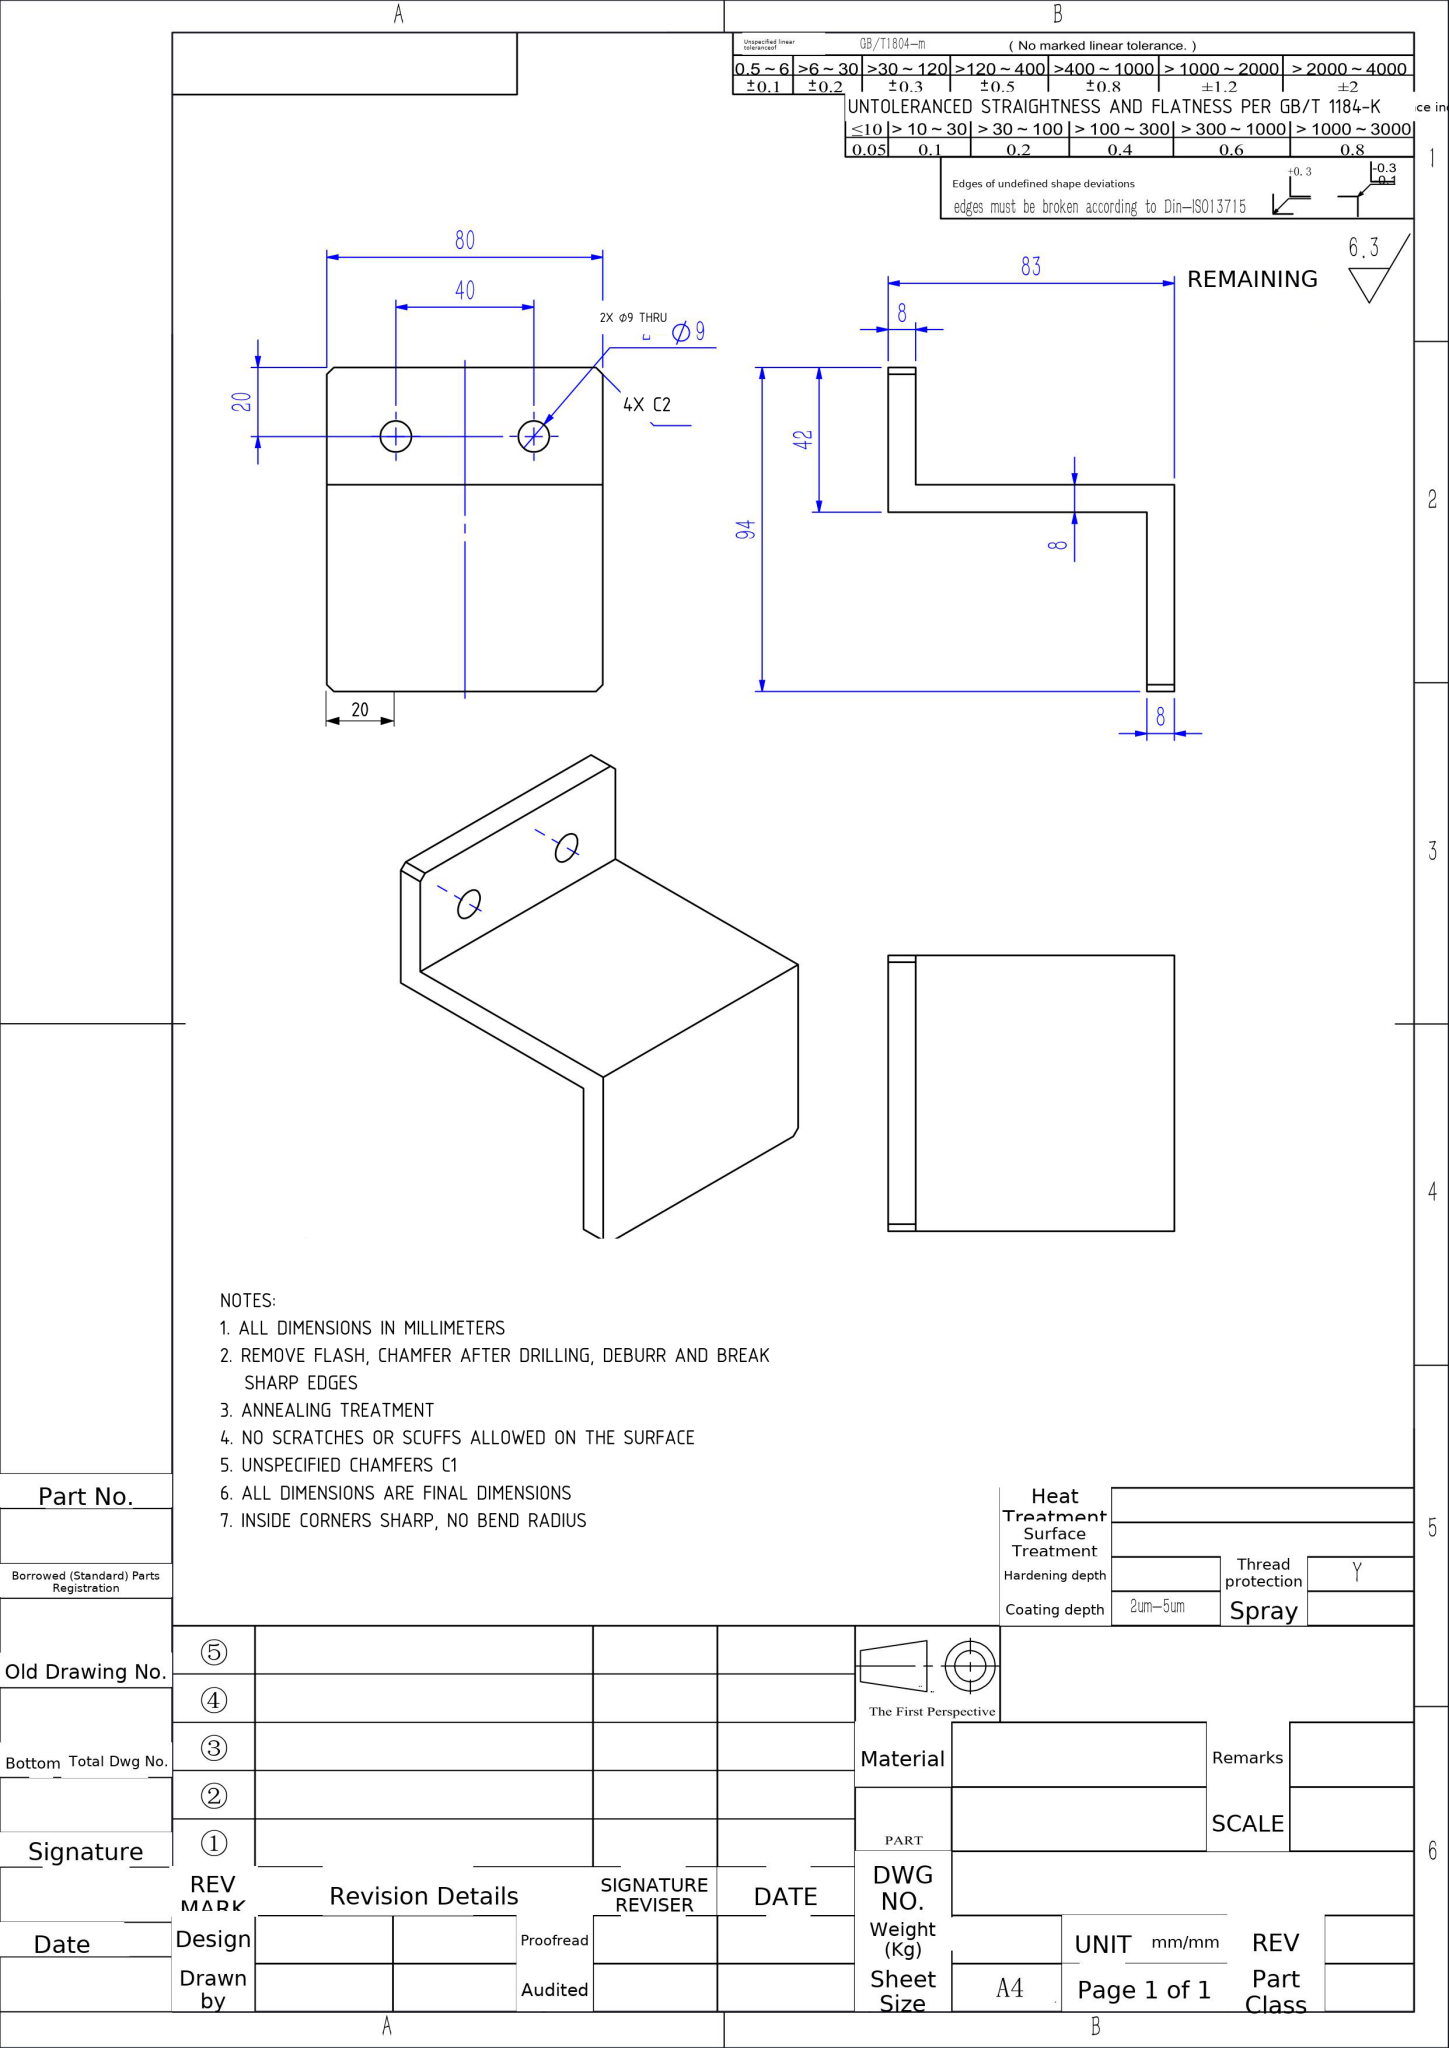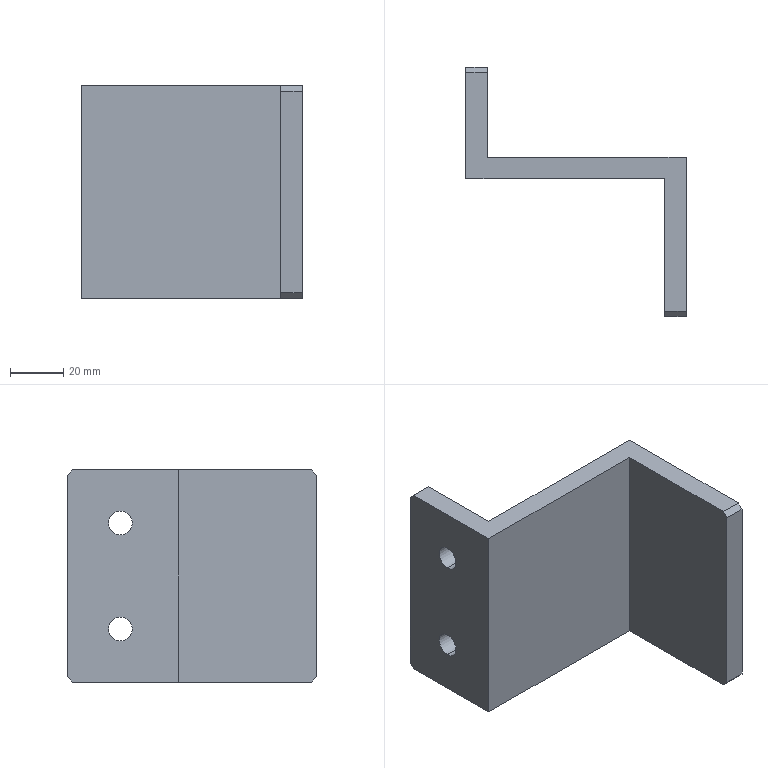Part | NX | mm | Chevron Notched Mounting Block | 1 solid | 18 faces | box 83 x 94 x 80 mm | volume 107078 mm3 | plane 14 | cylinder 4 | commonest cylinder face diameters 9 x4
STEP:
#1=COLOUR_RGB('',0.651,0.6196,0.5882);
#2=FILL_AREA_STYLE_COLOUR('',#1);
#3=FILL_AREA_STYLE('',(#2));
#4=SURFACE_STYLE_FILL_AREA(#3);
#5=SURFACE_SIDE_STYLE('',(#4));
#6=SURFACE_STYLE_USAGE(.BOTH.,#5);
#7=PRESENTATION_STYLE_ASSIGNMENT((#6));
#8=CARTESIAN_POINT('',(-75.,74.,24.5));
#9=VERTEX_POINT('',#8);
#10=CARTESIAN_POINT('',(-75.,74.,15.5));
#11=VERTEX_POINT('',#10);
#12=CARTESIAN_POINT('',(-75.,74.,20.));
#13=DIRECTION('',(1.,0.,-0.));
#14=DIRECTION('',(0.,0.,-1.));
#15=AXIS2_PLACEMENT_3D('',#12,#13,#14);
#16=CIRCLE('',#15,4.5);
#17=EDGE_CURVE('',#9,#11,#16,.T.);
#18=ORIENTED_EDGE('',*,*,#17,.F.);
#19=CARTESIAN_POINT('',(-67.,74.,24.5));
#20=VERTEX_POINT('',#19);
#21=CARTESIAN_POINT('',(-75.,74.,24.5));
#22=DIRECTION('',(1.,0.,-0.));
#23=VECTOR('',#22,1000.);
#24=LINE('',#21,#23);
#25=EDGE_CURVE('',#9,#20,#24,.T.);
#26=ORIENTED_EDGE('',*,*,#25,.T.);
#27=CARTESIAN_POINT('',(-67.,74.,15.5));
#28=VERTEX_POINT('',#27);
#29=CARTESIAN_POINT('',(-67.,74.,20.));
#30=DIRECTION('',(1.,0.,-0.));
#31=DIRECTION('',(0.,0.,-1.));
#32=AXIS2_PLACEMENT_3D('',#29,#30,#31);
#33=CIRCLE('',#32,4.5);
#34=EDGE_CURVE('',#20,#28,#33,.T.);
#35=ORIENTED_EDGE('',*,*,#34,.T.);
#36=CARTESIAN_POINT('',(-75.,74.,15.5));
#37=DIRECTION('',(1.,0.,-0.));
#38=VECTOR('',#37,1000.);
#39=LINE('',#36,#38);
#40=EDGE_CURVE('',#11,#28,#39,.T.);
#41=ORIENTED_EDGE('',*,*,#40,.F.);
#42=EDGE_LOOP('',(#18,#26,#35,#41));
#43=FACE_OUTER_BOUND('',#42,.T.);
#44=CARTESIAN_POINT('',(-75.,74.,20.));
#45=DIRECTION('',(1.,0.,-0.));
#46=DIRECTION('',(0.,0.,-1.));
#47=AXIS2_PLACEMENT_3D('',#44,#45,#46);
#48=CYLINDRICAL_SURFACE('',#47,4.5);
#49=ADVANCED_FACE('',(#43),#48,.F.);
#50=CARTESIAN_POINT('',(-75.,74.,64.5));
#51=VERTEX_POINT('',#50);
#52=CARTESIAN_POINT('',(-75.,74.,55.5));
#53=VERTEX_POINT('',#52);
#54=CARTESIAN_POINT('',(-75.,74.,60.));
#55=DIRECTION('',(1.,0.,-0.));
#56=DIRECTION('',(0.,0.,-1.));
#57=AXIS2_PLACEMENT_3D('',#54,#55,#56);
#58=CIRCLE('',#57,4.5);
#59=EDGE_CURVE('',#51,#53,#58,.T.);
#60=ORIENTED_EDGE('',*,*,#59,.F.);
#61=CARTESIAN_POINT('',(-67.,74.,64.5));
#62=VERTEX_POINT('',#61);
#63=CARTESIAN_POINT('',(-75.,74.,64.5));
#64=DIRECTION('',(1.,0.,-0.));
#65=VECTOR('',#64,1000.);
#66=LINE('',#63,#65);
#67=EDGE_CURVE('',#51,#62,#66,.T.);
#68=ORIENTED_EDGE('',*,*,#67,.T.);
#69=CARTESIAN_POINT('',(-67.,74.,55.5));
#70=VERTEX_POINT('',#69);
#71=CARTESIAN_POINT('',(-67.,74.,60.));
#72=DIRECTION('',(1.,0.,-0.));
#73=DIRECTION('',(0.,0.,-1.));
#74=AXIS2_PLACEMENT_3D('',#71,#72,#73);
#75=CIRCLE('',#74,4.5);
#76=EDGE_CURVE('',#62,#70,#75,.T.);
#77=ORIENTED_EDGE('',*,*,#76,.T.);
#78=CARTESIAN_POINT('',(-75.,74.,55.5));
#79=DIRECTION('',(1.,0.,-0.));
#80=VECTOR('',#79,1000.);
#81=LINE('',#78,#80);
#82=EDGE_CURVE('',#53,#70,#81,.T.);
#83=ORIENTED_EDGE('',*,*,#82,.F.);
#84=EDGE_LOOP('',(#60,#68,#77,#83));
#85=FACE_OUTER_BOUND('',#84,.T.);
#86=CARTESIAN_POINT('',(-75.,74.,60.));
#87=DIRECTION('',(1.,0.,-0.));
#88=DIRECTION('',(0.,0.,-1.));
#89=AXIS2_PLACEMENT_3D('',#86,#87,#88);
#90=CYLINDRICAL_SURFACE('',#89,4.5);
#91=ADVANCED_FACE('',(#85),#90,.F.);
#92=CARTESIAN_POINT('',(-67.,60.,80.));
#93=VERTEX_POINT('',#92);
#94=CARTESIAN_POINT('',(-67.,60.,0.));
#95=VERTEX_POINT('',#94);
#96=CARTESIAN_POINT('',(-67.,60.,0.));
#97=DIRECTION('',(-0.,0.,-1.));
#98=VECTOR('',#97,1000.);
#99=LINE('',#96,#98);
#100=EDGE_CURVE('',#93,#95,#99,.T.);
#101=ORIENTED_EDGE('',*,*,#100,.F.);
#102=CARTESIAN_POINT('',(8.,60.,80.));
#103=VERTEX_POINT('',#102);
#104=CARTESIAN_POINT('',(-75.,60.,80.));
#105=DIRECTION('',(-1.,0.,0.));
#106=VECTOR('',#105,1000.);
#107=LINE('',#104,#106);
#108=EDGE_CURVE('',#103,#93,#107,.T.);
#109=ORIENTED_EDGE('',*,*,#108,.F.);
#110=CARTESIAN_POINT('',(8.,60.,0.));
#111=VERTEX_POINT('',#110);
#112=CARTESIAN_POINT('',(8.,60.,80.));
#113=DIRECTION('',(0.,0.,-1.));
#114=VECTOR('',#113,1000.);
#115=LINE('',#112,#114);
#116=EDGE_CURVE('',#103,#111,#115,.T.);
#117=ORIENTED_EDGE('',*,*,#116,.T.);
#118=CARTESIAN_POINT('',(-75.,60.,0.));
#119=DIRECTION('',(-1.,0.,0.));
#120=VECTOR('',#119,1000.);
#121=LINE('',#118,#120);
#122=EDGE_CURVE('',#111,#95,#121,.T.);
#123=ORIENTED_EDGE('',*,*,#122,.T.);
#124=EDGE_LOOP('',(#101,#109,#117,#123));
#125=FACE_OUTER_BOUND('',#124,.T.);
#126=CARTESIAN_POINT('',(-75.,60.,80.));
#127=DIRECTION('',(0.,-1.,0.));
#128=DIRECTION('',(0.,0.,-1.));
#129=AXIS2_PLACEMENT_3D('',#126,#127,#128);
#130=PLANE('',#129);
#131=ADVANCED_FACE('',(#125),#130,.F.);
#132=CARTESIAN_POINT('',(8.,0.,78.));
#133=VERTEX_POINT('',#132);
#134=CARTESIAN_POINT('',(8.,0.,2.));
#135=VERTEX_POINT('',#134);
#136=CARTESIAN_POINT('',(8.,0.,80.));
#137=DIRECTION('',(0.,0.,-1.));
#138=VECTOR('',#137,1000.);
#139=LINE('',#136,#138);
#140=EDGE_CURVE('',#133,#135,#139,.T.);
#141=ORIENTED_EDGE('',*,*,#140,.F.);
#142=CARTESIAN_POINT('',(0.,0.,78.));
#143=VERTEX_POINT('',#142);
#144=CARTESIAN_POINT('',(8.,0.,78.));
#145=DIRECTION('',(-1.,0.,0.));
#146=VECTOR('',#145,1000.);
#147=LINE('',#144,#146);
#148=EDGE_CURVE('',#133,#143,#147,.T.);
#149=ORIENTED_EDGE('',*,*,#148,.T.);
#150=CARTESIAN_POINT('',(0.,0.,2.));
#151=VERTEX_POINT('',#150);
#152=CARTESIAN_POINT('',(0.,0.,80.));
#153=DIRECTION('',(0.,0.,-1.));
#154=VECTOR('',#153,1000.);
#155=LINE('',#152,#154);
#156=EDGE_CURVE('',#143,#151,#155,.T.);
#157=ORIENTED_EDGE('',*,*,#156,.T.);
#158=CARTESIAN_POINT('',(8.,0.,2.));
#159=DIRECTION('',(1.,0.,0.));
#160=VECTOR('',#159,1000.);
#161=LINE('',#158,#160);
#162=EDGE_CURVE('',#151,#135,#161,.T.);
#163=ORIENTED_EDGE('',*,*,#162,.T.);
#164=EDGE_LOOP('',(#141,#149,#157,#163));
#165=FACE_OUTER_BOUND('',#164,.T.);
#166=CARTESIAN_POINT('',(8.,0.,80.));
#167=DIRECTION('',(0.,1.,0.));
#168=DIRECTION('',(0.,0.,1.));
#169=AXIS2_PLACEMENT_3D('',#166,#167,#168);
#170=PLANE('',#169);
#171=ADVANCED_FACE('',(#165),#170,.F.);
#172=CARTESIAN_POINT('',(8.,2.,80.));
#173=VERTEX_POINT('',#172);
#174=CARTESIAN_POINT('',(8.,60.,80.));
#175=DIRECTION('',(-0.,1.,0.));
#176=VECTOR('',#175,1000.);
#177=LINE('',#174,#176);
#178=EDGE_CURVE('',#173,#103,#177,.T.);
#179=ORIENTED_EDGE('',*,*,#178,.F.);
#180=CARTESIAN_POINT('',(8.,2.,80.));
#181=DIRECTION('',(0.,-0.7071,-0.7071));
#182=VECTOR('',#181,1000.);
#183=LINE('',#180,#182);
#184=EDGE_CURVE('',#173,#133,#183,.T.);
#185=ORIENTED_EDGE('',*,*,#184,.T.);
#186=ORIENTED_EDGE('',*,*,#140,.T.);
#187=CARTESIAN_POINT('',(8.,2.,0.));
#188=VERTEX_POINT('',#187);
#189=CARTESIAN_POINT('',(8.,0.,2.));
#190=DIRECTION('',(-0.,0.7071,-0.7071));
#191=VECTOR('',#190,1000.);
#192=LINE('',#189,#191);
#193=EDGE_CURVE('',#135,#188,#192,.T.);
#194=ORIENTED_EDGE('',*,*,#193,.T.);
#195=CARTESIAN_POINT('',(8.,60.,0.));
#196=DIRECTION('',(-0.,1.,0.));
#197=VECTOR('',#196,1000.);
#198=LINE('',#195,#197);
#199=EDGE_CURVE('',#188,#111,#198,.T.);
#200=ORIENTED_EDGE('',*,*,#199,.T.);
#201=ORIENTED_EDGE('',*,*,#116,.F.);
#202=EDGE_LOOP('',(#179,#185,#186,#194,#200,#201));
#203=FACE_OUTER_BOUND('',#202,.T.);
#204=CARTESIAN_POINT('',(8.,60.,80.));
#205=DIRECTION('',(-1.,-0.,0.));
#206=DIRECTION('',(0.,-1.,0.));
#207=AXIS2_PLACEMENT_3D('',#204,#205,#206);
#208=PLANE('',#207);
#209=ADVANCED_FACE('',(#203),#208,.F.);
#210=CARTESIAN_POINT('',(-75.,74.,20.));
#211=DIRECTION('',(1.,0.,-0.));
#212=DIRECTION('',(0.,0.,-1.));
#213=AXIS2_PLACEMENT_3D('',#210,#211,#212);
#214=CIRCLE('',#213,4.5);
#215=EDGE_CURVE('',#11,#9,#214,.T.);
#216=ORIENTED_EDGE('',*,*,#215,.T.);
#217=ORIENTED_EDGE('',*,*,#17,.T.);
#218=EDGE_LOOP('',(#216,#217));
#219=FACE_BOUND('',#218,.T.);
#220=CARTESIAN_POINT('',(-75.,74.,60.));
#221=DIRECTION('',(1.,0.,-0.));
#222=DIRECTION('',(0.,0.,-1.));
#223=AXIS2_PLACEMENT_3D('',#220,#221,#222);
#224=CIRCLE('',#223,4.5);
#225=EDGE_CURVE('',#53,#51,#224,.T.);
#226=ORIENTED_EDGE('',*,*,#225,.T.);
#227=ORIENTED_EDGE('',*,*,#59,.T.);
#228=EDGE_LOOP('',(#226,#227));
#229=FACE_BOUND('',#228,.T.);
#230=CARTESIAN_POINT('',(-75.,94.,2.));
#231=VERTEX_POINT('',#230);
#232=CARTESIAN_POINT('',(-75.,94.,78.));
#233=VERTEX_POINT('',#232);
#234=CARTESIAN_POINT('',(-75.,94.,0.));
#235=DIRECTION('',(0.,0.,1.));
#236=VECTOR('',#235,1000.);
#237=LINE('',#234,#236);
#238=EDGE_CURVE('',#231,#233,#237,.T.);
#239=ORIENTED_EDGE('',*,*,#238,.F.);
#240=CARTESIAN_POINT('',(-75.,92.,0.));
#241=VERTEX_POINT('',#240);
#242=CARTESIAN_POINT('',(-75.,94.,2.));
#243=DIRECTION('',(0.,-0.7071,-0.7071));
#244=VECTOR('',#243,1000.);
#245=LINE('',#242,#244);
#246=EDGE_CURVE('',#231,#241,#245,.T.);
#247=ORIENTED_EDGE('',*,*,#246,.T.);
#248=CARTESIAN_POINT('',(-75.,52.,0.));
#249=VERTEX_POINT('',#248);
#250=CARTESIAN_POINT('',(-75.,52.,0.));
#251=DIRECTION('',(0.,-1.,0.));
#252=VECTOR('',#251,1000.);
#253=LINE('',#250,#252);
#254=EDGE_CURVE('',#241,#249,#253,.T.);
#255=ORIENTED_EDGE('',*,*,#254,.T.);
#256=CARTESIAN_POINT('',(-75.,52.,80.));
#257=VERTEX_POINT('',#256);
#258=CARTESIAN_POINT('',(-75.,52.,80.));
#259=DIRECTION('',(0.,0.,-1.));
#260=VECTOR('',#259,1000.);
#261=LINE('',#258,#260);
#262=EDGE_CURVE('',#257,#249,#261,.T.);
#263=ORIENTED_EDGE('',*,*,#262,.F.);
#264=CARTESIAN_POINT('',(-75.,92.,80.));
#265=VERTEX_POINT('',#264);
#266=CARTESIAN_POINT('',(-75.,52.,80.));
#267=DIRECTION('',(0.,-1.,0.));
#268=VECTOR('',#267,1000.);
#269=LINE('',#266,#268);
#270=EDGE_CURVE('',#265,#257,#269,.T.);
#271=ORIENTED_EDGE('',*,*,#270,.F.);
#272=CARTESIAN_POINT('',(-75.,94.,78.));
#273=DIRECTION('',(0.,0.7071,-0.7071));
#274=VECTOR('',#273,1000.);
#275=LINE('',#272,#274);
#276=EDGE_CURVE('',#265,#233,#275,.T.);
#277=ORIENTED_EDGE('',*,*,#276,.T.);
#278=EDGE_LOOP('',(#239,#247,#255,#263,#271,#277));
#279=FACE_OUTER_BOUND('',#278,.T.);
#280=CARTESIAN_POINT('',(-75.,52.,80.));
#281=DIRECTION('',(1.,0.,0.));
#282=DIRECTION('',(0.,0.,-1.));
#283=AXIS2_PLACEMENT_3D('',#280,#281,#282);
#284=PLANE('',#283);
#285=ADVANCED_FACE('',(#219,#229,#279),#284,.F.);
#286=CARTESIAN_POINT('',(0.,52.,0.));
#287=VERTEX_POINT('',#286);
#288=CARTESIAN_POINT('',(0.,52.,0.));
#289=DIRECTION('',(1.,0.,0.));
#290=VECTOR('',#289,1000.);
#291=LINE('',#288,#290);
#292=EDGE_CURVE('',#249,#287,#291,.T.);
#293=ORIENTED_EDGE('',*,*,#292,.T.);
#294=CARTESIAN_POINT('',(0.,52.,80.));
#295=VERTEX_POINT('',#294);
#296=CARTESIAN_POINT('',(0.,52.,80.));
#297=DIRECTION('',(0.,0.,-1.));
#298=VECTOR('',#297,1000.);
#299=LINE('',#296,#298);
#300=EDGE_CURVE('',#295,#287,#299,.T.);
#301=ORIENTED_EDGE('',*,*,#300,.F.);
#302=CARTESIAN_POINT('',(0.,52.,80.));
#303=DIRECTION('',(1.,0.,0.));
#304=VECTOR('',#303,1000.);
#305=LINE('',#302,#304);
#306=EDGE_CURVE('',#257,#295,#305,.T.);
#307=ORIENTED_EDGE('',*,*,#306,.F.);
#308=ORIENTED_EDGE('',*,*,#262,.T.);
#309=EDGE_LOOP('',(#293,#301,#307,#308));
#310=FACE_OUTER_BOUND('',#309,.T.);
#311=CARTESIAN_POINT('',(0.,52.,80.));
#312=DIRECTION('',(-0.,1.,0.));
#313=DIRECTION('',(-1.,-0.,0.));
#314=AXIS2_PLACEMENT_3D('',#311,#312,#313);
#315=PLANE('',#314);
#316=ADVANCED_FACE('',(#310),#315,.F.);
#317=ORIENTED_EDGE('',*,*,#156,.F.);
#318=CARTESIAN_POINT('',(0.,2.,80.));
#319=VERTEX_POINT('',#318);
#320=CARTESIAN_POINT('',(0.,2.,80.));
#321=DIRECTION('',(0.,0.7071,0.7071));
#322=VECTOR('',#321,1000.);
#323=LINE('',#320,#322);
#324=EDGE_CURVE('',#143,#319,#323,.T.);
#325=ORIENTED_EDGE('',*,*,#324,.T.);
#326=CARTESIAN_POINT('',(0.,0.,80.));
#327=DIRECTION('',(0.,-1.,0.));
#328=VECTOR('',#327,1000.);
#329=LINE('',#326,#328);
#330=EDGE_CURVE('',#295,#319,#329,.T.);
#331=ORIENTED_EDGE('',*,*,#330,.F.);
#332=ORIENTED_EDGE('',*,*,#300,.T.);
#333=CARTESIAN_POINT('',(0.,2.,0.));
#334=VERTEX_POINT('',#333);
#335=CARTESIAN_POINT('',(0.,0.,0.));
#336=DIRECTION('',(0.,-1.,0.));
#337=VECTOR('',#336,1000.);
#338=LINE('',#335,#337);
#339=EDGE_CURVE('',#287,#334,#338,.T.);
#340=ORIENTED_EDGE('',*,*,#339,.T.);
#341=CARTESIAN_POINT('',(0.,0.,2.));
#342=DIRECTION('',(0.,-0.7071,0.7071));
#343=VECTOR('',#342,1000.);
#344=LINE('',#341,#343);
#345=EDGE_CURVE('',#334,#151,#344,.T.);
#346=ORIENTED_EDGE('',*,*,#345,.T.);
#347=EDGE_LOOP('',(#317,#325,#331,#332,#340,#346));
#348=FACE_OUTER_BOUND('',#347,.T.);
#349=CARTESIAN_POINT('',(0.,0.,80.));
#350=DIRECTION('',(1.,0.,0.));
#351=DIRECTION('',(0.,0.,-1.));
#352=AXIS2_PLACEMENT_3D('',#349,#350,#351);
#353=PLANE('',#352);
#354=ADVANCED_FACE('',(#348),#353,.F.);
#355=ORIENTED_EDGE('',*,*,#330,.T.);
#356=CARTESIAN_POINT('',(0.,2.,80.));
#357=DIRECTION('',(1.,0.,0.));
#358=VECTOR('',#357,1000.);
#359=LINE('',#356,#358);
#360=EDGE_CURVE('',#319,#173,#359,.T.);
#361=ORIENTED_EDGE('',*,*,#360,.T.);
#362=ORIENTED_EDGE('',*,*,#178,.T.);
#363=ORIENTED_EDGE('',*,*,#108,.T.);
#364=CARTESIAN_POINT('',(-67.,92.,80.));
#365=VERTEX_POINT('',#364);
#366=CARTESIAN_POINT('',(-67.,94.,80.));
#367=DIRECTION('',(0.,-1.,0.));
#368=VECTOR('',#367,1000.);
#369=LINE('',#366,#368);
#370=EDGE_CURVE('',#365,#93,#369,.T.);
#371=ORIENTED_EDGE('',*,*,#370,.F.);
#372=CARTESIAN_POINT('',(-75.,92.,80.));
#373=DIRECTION('',(-1.,0.,0.));
#374=VECTOR('',#373,1000.);
#375=LINE('',#372,#374);
#376=EDGE_CURVE('',#365,#265,#375,.T.);
#377=ORIENTED_EDGE('',*,*,#376,.T.);
#378=ORIENTED_EDGE('',*,*,#270,.T.);
#379=ORIENTED_EDGE('',*,*,#306,.T.);
#380=EDGE_LOOP('',(#355,#361,#362,#363,#371,#377,#378,#379));
#381=FACE_OUTER_BOUND('',#380,.T.);
#382=CARTESIAN_POINT('',(0.,0.,80.));
#383=DIRECTION('',(0.,0.,-1.));
#384=DIRECTION('',(-1.,0.,0.));
#385=AXIS2_PLACEMENT_3D('',#382,#383,#384);
#386=PLANE('',#385);
#387=ADVANCED_FACE('',(#381),#386,.F.);
#388=ORIENTED_EDGE('',*,*,#199,.F.);
#389=CARTESIAN_POINT('',(0.,2.,0.));
#390=DIRECTION('',(-1.,0.,0.));
#391=VECTOR('',#390,1000.);
#392=LINE('',#389,#391);
#393=EDGE_CURVE('',#188,#334,#392,.T.);
#394=ORIENTED_EDGE('',*,*,#393,.T.);
#395=ORIENTED_EDGE('',*,*,#339,.F.);
#396=ORIENTED_EDGE('',*,*,#292,.F.);
#397=ORIENTED_EDGE('',*,*,#254,.F.);
#398=CARTESIAN_POINT('',(-67.,92.,0.));
#399=VERTEX_POINT('',#398);
#400=CARTESIAN_POINT('',(0.,92.,0.));
#401=DIRECTION('',(1.,0.,0.));
#402=VECTOR('',#401,1000.);
#403=LINE('',#400,#402);
#404=EDGE_CURVE('',#241,#399,#403,.T.);
#405=ORIENTED_EDGE('',*,*,#404,.T.);
#406=CARTESIAN_POINT('',(-67.,94.,0.));
#407=DIRECTION('',(0.,-1.,0.));
#408=VECTOR('',#407,1000.);
#409=LINE('',#406,#408);
#410=EDGE_CURVE('',#399,#95,#409,.T.);
#411=ORIENTED_EDGE('',*,*,#410,.T.);
#412=ORIENTED_EDGE('',*,*,#122,.F.);
#413=EDGE_LOOP('',(#388,#394,#395,#396,#397,#405,#411,#412));
#414=FACE_OUTER_BOUND('',#413,.T.);
#415=CARTESIAN_POINT('',(0.,0.,0.));
#416=DIRECTION('',(0.,0.,-1.));
#417=DIRECTION('',(-1.,0.,0.));
#418=AXIS2_PLACEMENT_3D('',#415,#416,#417);
#419=PLANE('',#418);
#420=ADVANCED_FACE('',(#414),#419,.T.);
#421=CARTESIAN_POINT('',(-67.,74.,20.));
#422=DIRECTION('',(1.,0.,-0.));
#423=DIRECTION('',(0.,0.,-1.));
#424=AXIS2_PLACEMENT_3D('',#421,#422,#423);
#425=CIRCLE('',#424,4.5);
#426=EDGE_CURVE('',#28,#20,#425,.T.);
#427=ORIENTED_EDGE('',*,*,#426,.F.);
#428=ORIENTED_EDGE('',*,*,#34,.F.);
#429=EDGE_LOOP('',(#427,#428));
#430=FACE_BOUND('',#429,.T.);
#431=CARTESIAN_POINT('',(-67.,74.,60.));
#432=DIRECTION('',(1.,0.,-0.));
#433=DIRECTION('',(0.,0.,-1.));
#434=AXIS2_PLACEMENT_3D('',#431,#432,#433);
#435=CIRCLE('',#434,4.5);
#436=EDGE_CURVE('',#70,#62,#435,.T.);
#437=ORIENTED_EDGE('',*,*,#436,.F.);
#438=ORIENTED_EDGE('',*,*,#76,.F.);
#439=EDGE_LOOP('',(#437,#438));
#440=FACE_BOUND('',#439,.T.);
#441=ORIENTED_EDGE('',*,*,#410,.F.);
#442=CARTESIAN_POINT('',(-67.,94.,2.));
#443=VERTEX_POINT('',#442);
#444=CARTESIAN_POINT('',(-67.,94.,2.));
#445=DIRECTION('',(0.,0.7071,0.7071));
#446=VECTOR('',#445,1000.);
#447=LINE('',#444,#446);
#448=EDGE_CURVE('',#399,#443,#447,.T.);
#449=ORIENTED_EDGE('',*,*,#448,.T.);
#450=CARTESIAN_POINT('',(-67.,94.,78.));
#451=VERTEX_POINT('',#450);
#452=CARTESIAN_POINT('',(-67.,94.,0.));
#453=DIRECTION('',(-0.,0.,-1.));
#454=VECTOR('',#453,1000.);
#455=LINE('',#452,#454);
#456=EDGE_CURVE('',#451,#443,#455,.T.);
#457=ORIENTED_EDGE('',*,*,#456,.F.);
#458=CARTESIAN_POINT('',(-67.,94.,78.));
#459=DIRECTION('',(0.,-0.7071,0.7071));
#460=VECTOR('',#459,1000.);
#461=LINE('',#458,#460);
#462=EDGE_CURVE('',#451,#365,#461,.T.);
#463=ORIENTED_EDGE('',*,*,#462,.T.);
#464=ORIENTED_EDGE('',*,*,#370,.T.);
#465=ORIENTED_EDGE('',*,*,#100,.T.);
#466=EDGE_LOOP('',(#441,#449,#457,#463,#464,#465));
#467=FACE_OUTER_BOUND('',#466,.T.);
#468=CARTESIAN_POINT('',(-67.,94.,0.));
#469=DIRECTION('',(-1.,0.,0.));
#470=DIRECTION('',(0.,0.,1.));
#471=AXIS2_PLACEMENT_3D('',#468,#469,#470);
#472=PLANE('',#471);
#473=ADVANCED_FACE('',(#430,#440,#467),#472,.F.);
#474=ORIENTED_EDGE('',*,*,#456,.T.);
#475=CARTESIAN_POINT('',(0.,94.,2.));
#476=DIRECTION('',(-1.,0.,0.));
#477=VECTOR('',#476,1000.);
#478=LINE('',#475,#477);
#479=EDGE_CURVE('',#443,#231,#478,.T.);
#480=ORIENTED_EDGE('',*,*,#479,.T.);
#481=ORIENTED_EDGE('',*,*,#238,.T.);
#482=CARTESIAN_POINT('',(-67.,94.,78.));
#483=DIRECTION('',(1.,0.,0.));
#484=VECTOR('',#483,1000.);
#485=LINE('',#482,#484);
#486=EDGE_CURVE('',#233,#451,#485,.T.);
#487=ORIENTED_EDGE('',*,*,#486,.T.);
#488=EDGE_LOOP('',(#474,#480,#481,#487));
#489=FACE_OUTER_BOUND('',#488,.T.);
#490=CARTESIAN_POINT('',(0.,94.,0.));
#491=DIRECTION('',(0.,1.,0.));
#492=DIRECTION('',(0.,0.,1.));
#493=AXIS2_PLACEMENT_3D('',#490,#491,#492);
#494=PLANE('',#493);
#495=ADVANCED_FACE('',(#489),#494,.T.);
#496=ORIENTED_EDGE('',*,*,#67,.F.);
#497=ORIENTED_EDGE('',*,*,#225,.F.);
#498=ORIENTED_EDGE('',*,*,#82,.T.);
#499=ORIENTED_EDGE('',*,*,#436,.T.);
#500=EDGE_LOOP('',(#496,#497,#498,#499));
#501=FACE_OUTER_BOUND('',#500,.T.);
#502=CARTESIAN_POINT('',(-75.,74.,60.));
#503=DIRECTION('',(1.,0.,-0.));
#504=DIRECTION('',(0.,0.,-1.));
#505=AXIS2_PLACEMENT_3D('',#502,#503,#504);
#506=CYLINDRICAL_SURFACE('',#505,4.5);
#507=ADVANCED_FACE('',(#501),#506,.F.);
#508=ORIENTED_EDGE('',*,*,#25,.F.);
#509=ORIENTED_EDGE('',*,*,#215,.F.);
#510=ORIENTED_EDGE('',*,*,#40,.T.);
#511=ORIENTED_EDGE('',*,*,#426,.T.);
#512=EDGE_LOOP('',(#508,#509,#510,#511));
#513=FACE_OUTER_BOUND('',#512,.T.);
#514=CARTESIAN_POINT('',(-75.,74.,20.));
#515=DIRECTION('',(1.,0.,-0.));
#516=DIRECTION('',(0.,0.,-1.));
#517=AXIS2_PLACEMENT_3D('',#514,#515,#516);
#518=CYLINDRICAL_SURFACE('',#517,4.5);
#519=ADVANCED_FACE('',(#513),#518,.F.);
#520=ORIENTED_EDGE('',*,*,#324,.F.);
#521=ORIENTED_EDGE('',*,*,#148,.F.);
#522=ORIENTED_EDGE('',*,*,#184,.F.);
#523=ORIENTED_EDGE('',*,*,#360,.F.);
#524=EDGE_LOOP('',(#520,#521,#522,#523));
#525=FACE_OUTER_BOUND('',#524,.T.);
#526=CARTESIAN_POINT('',(0.,2.,80.));
#527=DIRECTION('',(0.,0.7071,-0.7071));
#528=DIRECTION('',(1.,0.,0.));
#529=AXIS2_PLACEMENT_3D('',#526,#527,#528);
#530=PLANE('',#529);
#531=ADVANCED_FACE('',(#525),#530,.F.);
#532=ORIENTED_EDGE('',*,*,#345,.F.);
#533=ORIENTED_EDGE('',*,*,#393,.F.);
#534=ORIENTED_EDGE('',*,*,#193,.F.);
#535=ORIENTED_EDGE('',*,*,#162,.F.);
#536=EDGE_LOOP('',(#532,#533,#534,#535));
#537=FACE_OUTER_BOUND('',#536,.T.);
#538=CARTESIAN_POINT('',(8.,0.,2.));
#539=DIRECTION('',(0.,-0.7071,-0.7071));
#540=DIRECTION('',(-1.,0.,0.));
#541=AXIS2_PLACEMENT_3D('',#538,#539,#540);
#542=PLANE('',#541);
#543=ADVANCED_FACE('',(#537),#542,.T.);
#544=ORIENTED_EDGE('',*,*,#448,.F.);
#545=ORIENTED_EDGE('',*,*,#404,.F.);
#546=ORIENTED_EDGE('',*,*,#246,.F.);
#547=ORIENTED_EDGE('',*,*,#479,.F.);
#548=EDGE_LOOP('',(#544,#545,#546,#547));
#549=FACE_OUTER_BOUND('',#548,.T.);
#550=CARTESIAN_POINT('',(0.,94.,2.));
#551=DIRECTION('',(0.,-0.7071,0.7071));
#552=DIRECTION('',(-1.,0.,0.));
#553=AXIS2_PLACEMENT_3D('',#550,#551,#552);
#554=PLANE('',#553);
#555=ADVANCED_FACE('',(#549),#554,.F.);
#556=ORIENTED_EDGE('',*,*,#276,.F.);
#557=ORIENTED_EDGE('',*,*,#376,.F.);
#558=ORIENTED_EDGE('',*,*,#462,.F.);
#559=ORIENTED_EDGE('',*,*,#486,.F.);
#560=EDGE_LOOP('',(#556,#557,#558,#559));
#561=FACE_OUTER_BOUND('',#560,.T.);
#562=CARTESIAN_POINT('',(0.,94.,78.));
#563=DIRECTION('',(0.,0.7071,0.7071));
#564=DIRECTION('',(-1.,0.,0.));
#565=AXIS2_PLACEMENT_3D('',#562,#563,#564);
#566=PLANE('',#565);
#567=ADVANCED_FACE('',(#561),#566,.T.);
#568=CLOSED_SHELL('',(#49,#91,#131,#171,#209,#285,#316,#354,#387,#420,#473,#495,#507,#519,#531,#543,#555,#567));
#569=MANIFOLD_SOLID_BREP('',#568);
#570=CARTESIAN_POINT('',(0.,0.,0.));
#571=DIRECTION('',(0.,0.,1.));
#572=DIRECTION('',(1.,0.,0.));
#573=AXIS2_PLACEMENT_3D('',#570,#571,#572);
#574=(LENGTH_UNIT()NAMED_UNIT(*)SI_UNIT(.MILLI.,.METRE.));
#575=UNCERTAINTY_MEASURE_WITH_UNIT(LENGTH_MEASURE(0.00001),#574,'','');
#576=(NAMED_UNIT(*)PLANE_ANGLE_UNIT()SI_UNIT($,.RADIAN.));
#577=(NAMED_UNIT(*)SI_UNIT($,.STERADIAN.)SOLID_ANGLE_UNIT());
#578=(GEOMETRIC_REPRESENTATION_CONTEXT(3)GLOBAL_UNCERTAINTY_ASSIGNED_CONTEXT((#575))GLOBAL_UNIT_ASSIGNED_CONTEXT((#574,#576,#577))REPRESENTATION_CONTEXT('',''));
#579=ADVANCED_BREP_SHAPE_REPRESENTATION('',(#569,#573),#578);
#580=STYLED_ITEM('',(#7),#579);
#581=PRESENTATION_LAYER_ASSIGNMENT('','',(#580));
#582=(LENGTH_UNIT()NAMED_UNIT(*)SI_UNIT(.MILLI.,.METRE.));
#583=UNCERTAINTY_MEASURE_WITH_UNIT(LENGTH_MEASURE(0.00001),#582,'','');
#584=(NAMED_UNIT(*)PLANE_ANGLE_UNIT()SI_UNIT($,.RADIAN.));
#585=(NAMED_UNIT(*)SI_UNIT($,.STERADIAN.)SOLID_ANGLE_UNIT());
#586=(GEOMETRIC_REPRESENTATION_CONTEXT(3)GLOBAL_UNCERTAINTY_ASSIGNED_CONTEXT((#583))GLOBAL_UNIT_ASSIGNED_CONTEXT((#582,#584,#585))REPRESENTATION_CONTEXT('',''));
#587=MECHANICAL_DESIGN_GEOMETRIC_PRESENTATION_REPRESENTATION('',(#580),#586);
#588=COLOUR_RGB('',0.651,0.6196,0.5882);
#589=FILL_AREA_STYLE_COLOUR('',#588);
#590=FILL_AREA_STYLE('',(#589));
#591=SURFACE_STYLE_FILL_AREA(#590);
#592=SURFACE_SIDE_STYLE('',(#591));
#593=SURFACE_STYLE_USAGE(.BOTH.,#592);
#594=PRESENTATION_STYLE_ASSIGNMENT((#593));
#595=STYLED_ITEM('',(#594),#569);
#596=(LENGTH_UNIT()NAMED_UNIT(*)SI_UNIT(.MILLI.,.METRE.));
#597=UNCERTAINTY_MEASURE_WITH_UNIT(LENGTH_MEASURE(0.00001),#596,'','');
#598=(NAMED_UNIT(*)PLANE_ANGLE_UNIT()SI_UNIT($,.RADIAN.));
#599=(NAMED_UNIT(*)SI_UNIT($,.STERADIAN.)SOLID_ANGLE_UNIT());
#600=(GEOMETRIC_REPRESENTATION_CONTEXT(3)GLOBAL_UNCERTAINTY_ASSIGNED_CONTEXT((#597))GLOBAL_UNIT_ASSIGNED_CONTEXT((#596,#598,#599))REPRESENTATION_CONTEXT('',''));
#601=MECHANICAL_DESIGN_GEOMETRIC_PRESENTATION_REPRESENTATION('',(#595),#600);
#602=PRESENTATION_LAYER_ASSIGNMENT('','',(#595));